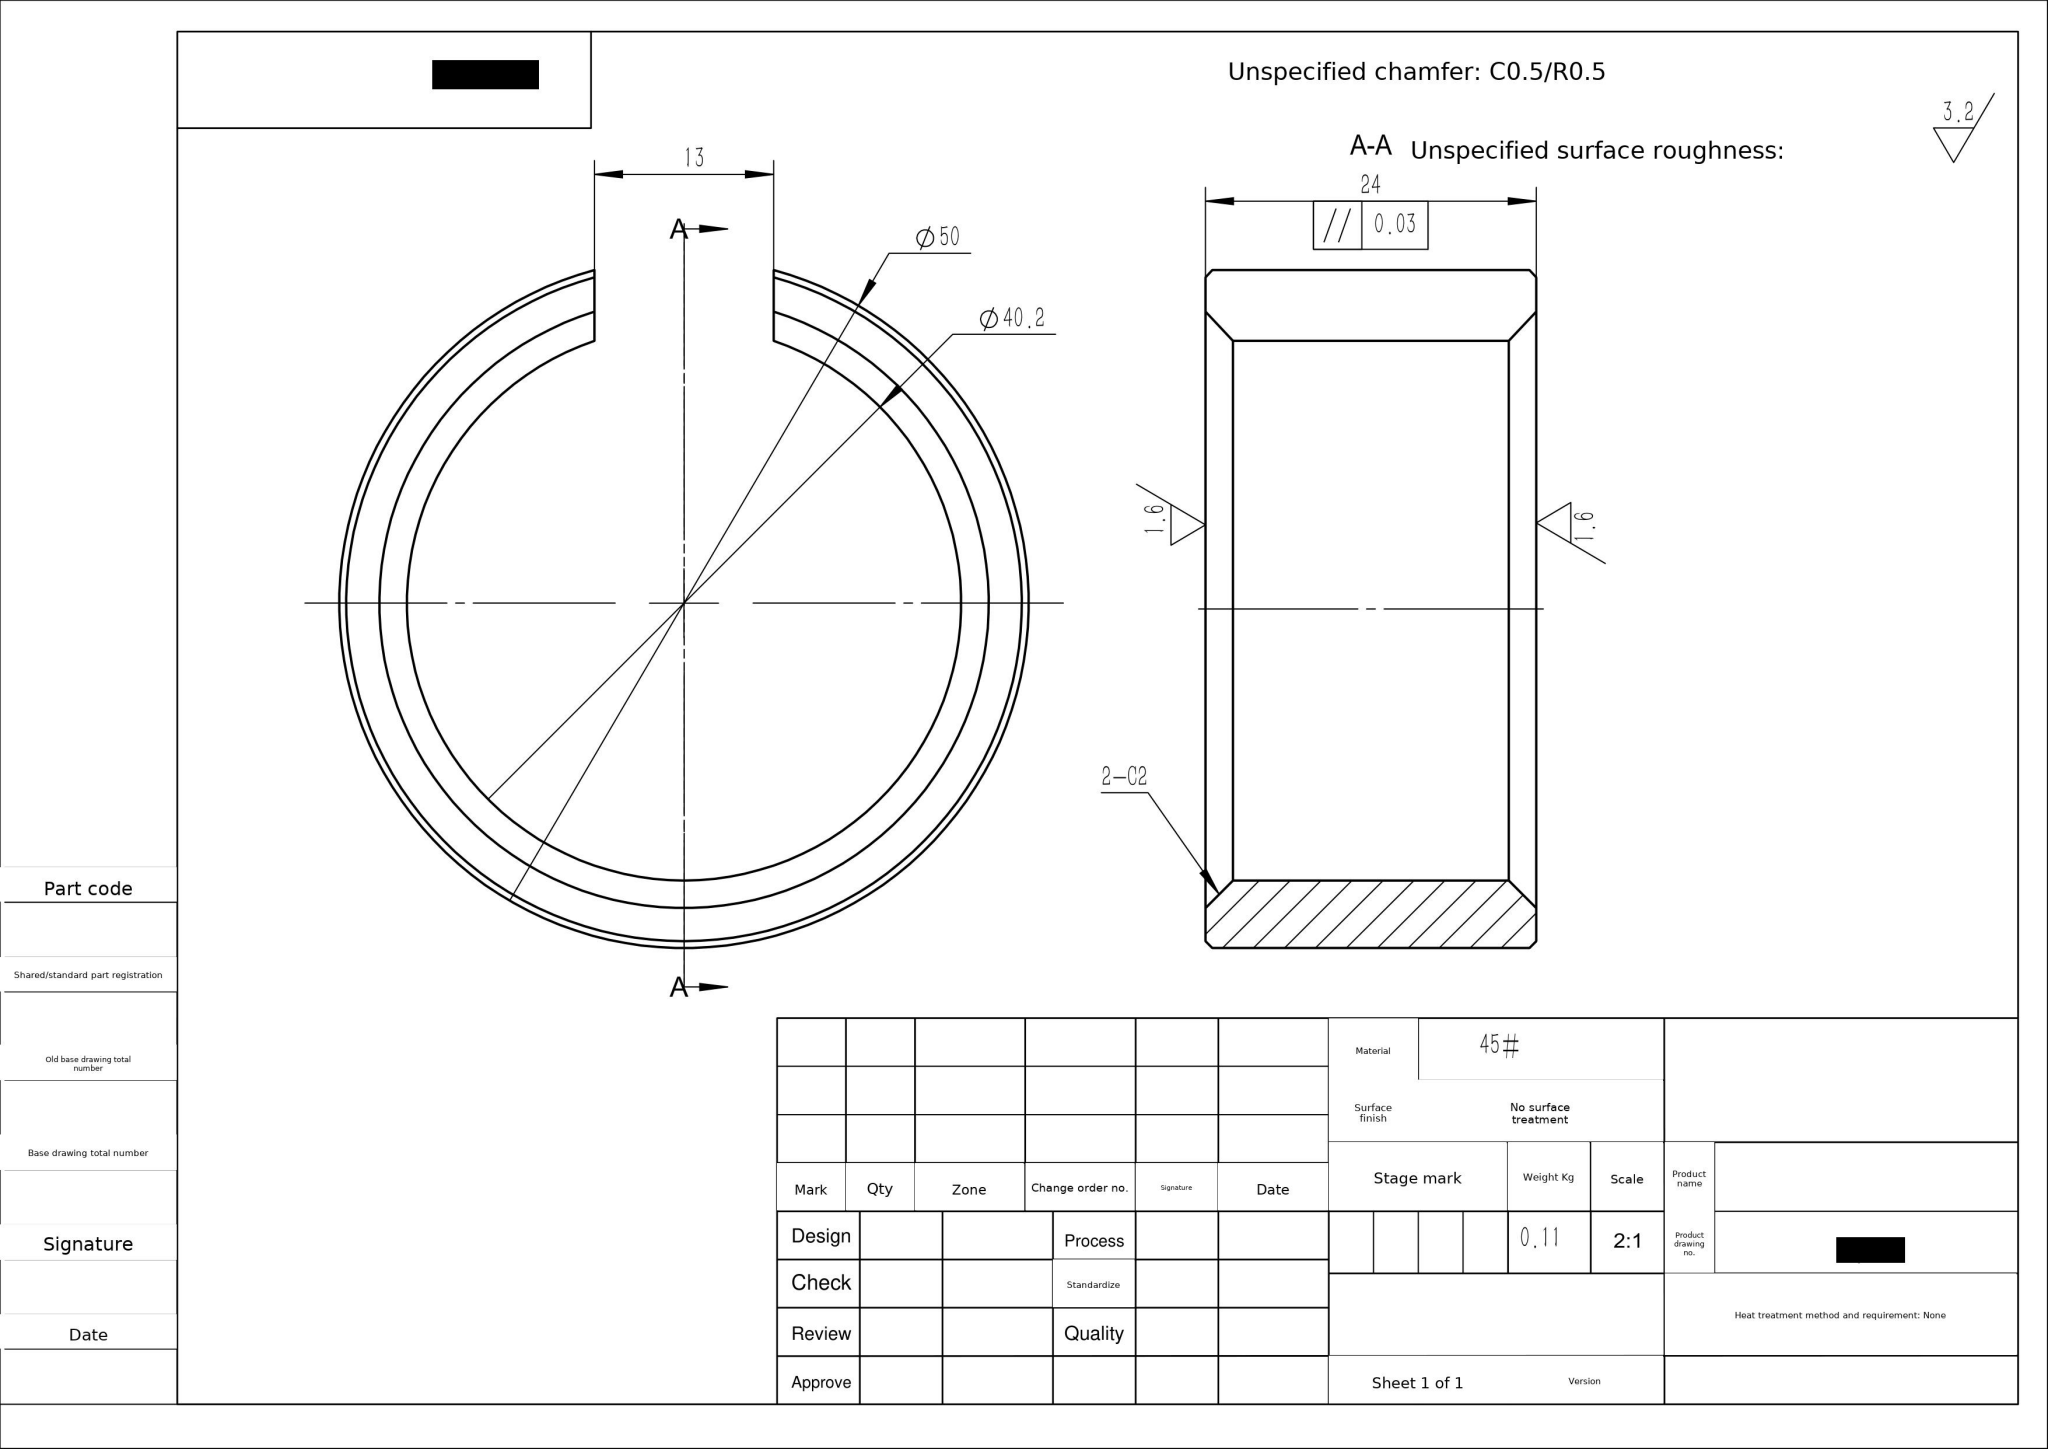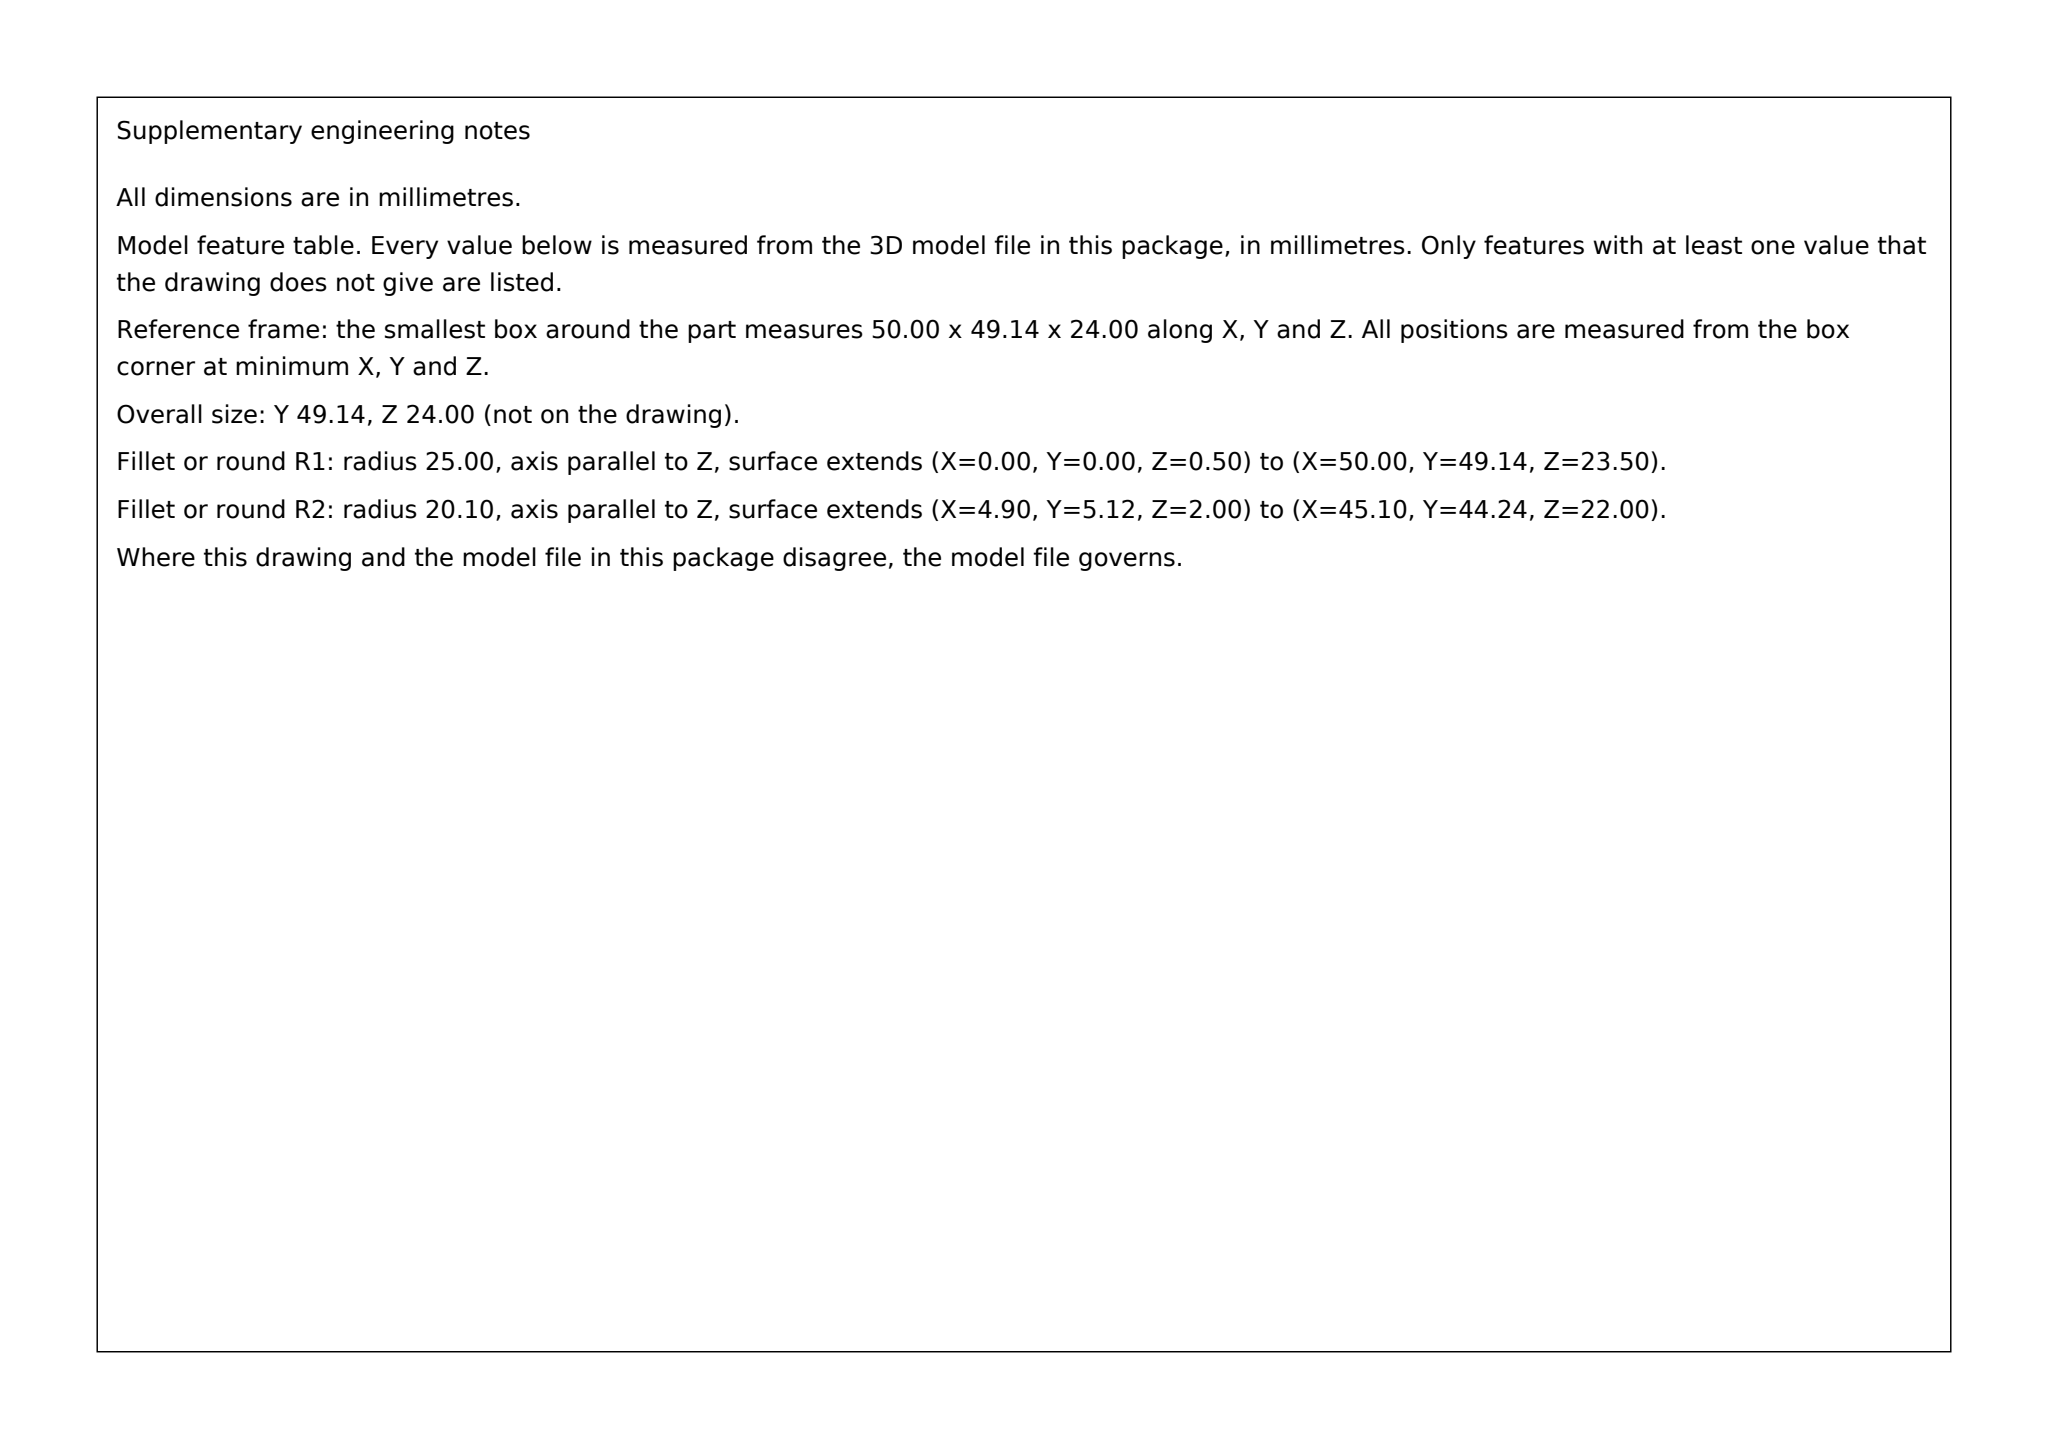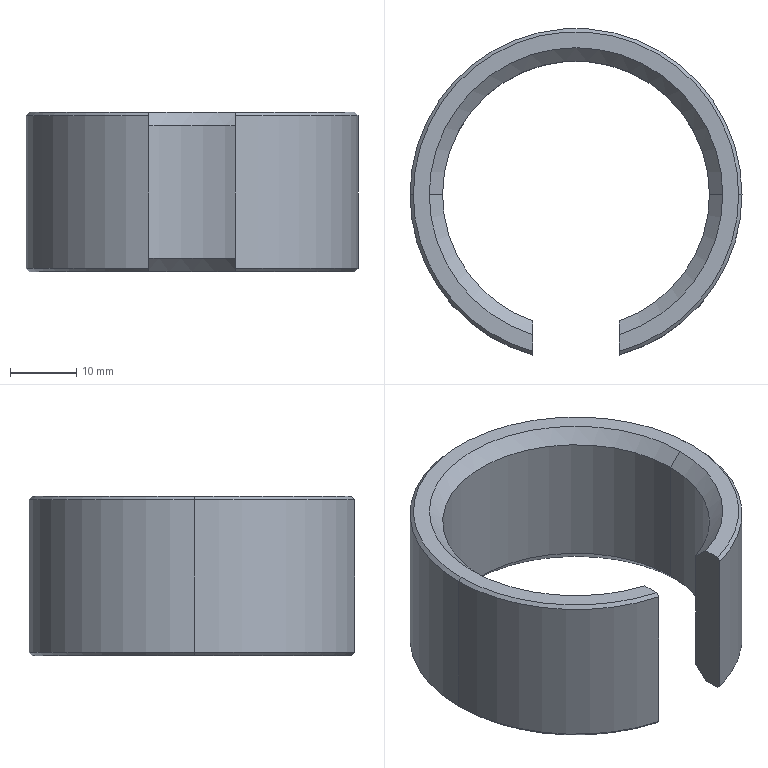Part | SolidWorks | mm | material 45# | 1 solid | 22 faces | box 50 x 49.14 x 24 mm | volume 14606 mm3 | cone 12 | cylinder 6 | plane 4 | commonest cylinder face diameters 40.2 x3 50 x3
build123d program:
from build123d import *

# Parameters (mm, degrees)
SKETCH1_R           = 25
SKETCH1_R_2         = 20.1
BOSS_EXTRUDE1_DEPTH = 24
SKETCH2_W           = 13
SKETCH2_H           = 27.854
CUT_EXTRUDE1_DEPTH  = 43.732
CHAMFER1_SIZE       = 0.5
CHAMFER2_SIZE       = 2


with BuildPart() as part:
    # Sketch1 → Boss-Extrude1 (new body)
    with BuildSketch(Plane.XY):
        Circle(SKETCH1_R)
        Circle(SKETCH1_R_2, mode=Mode.SUBTRACT)
    extrude(amount=BOSS_EXTRUDE1_DEPTH)

    # Sketch2 → Cut-Extrude1 (cut, through all)
    with BuildSketch(Plane(origin=(0, 0, 0), x_dir=(-1, 0, 0), z_dir=(0, 0, -1))):
        with Locations((0, -13.927)):
            Rectangle(SKETCH2_W, SKETCH2_H)
    extrude(amount=-CUT_EXTRUDE1_DEPTH, mode=Mode.SUBTRACT)

    # Chamfer1
    chamfer1_edges = [part.edges().sort_by_distance(p)[0] for p in [
        (0, 25, 24),
        (0, 25, 0),
    ]]
    chamfer(chamfer1_edges, length=CHAMFER1_SIZE)

    # Chamfer2
    chamfer2_edges = [part.edges().sort_by_distance(p)[0] for p in [
        (0, 20.1, 0),
        (0, 20.1, 24),
    ]]
    chamfer(chamfer2_edges, length=CHAMFER2_SIZE)


solid = part.part